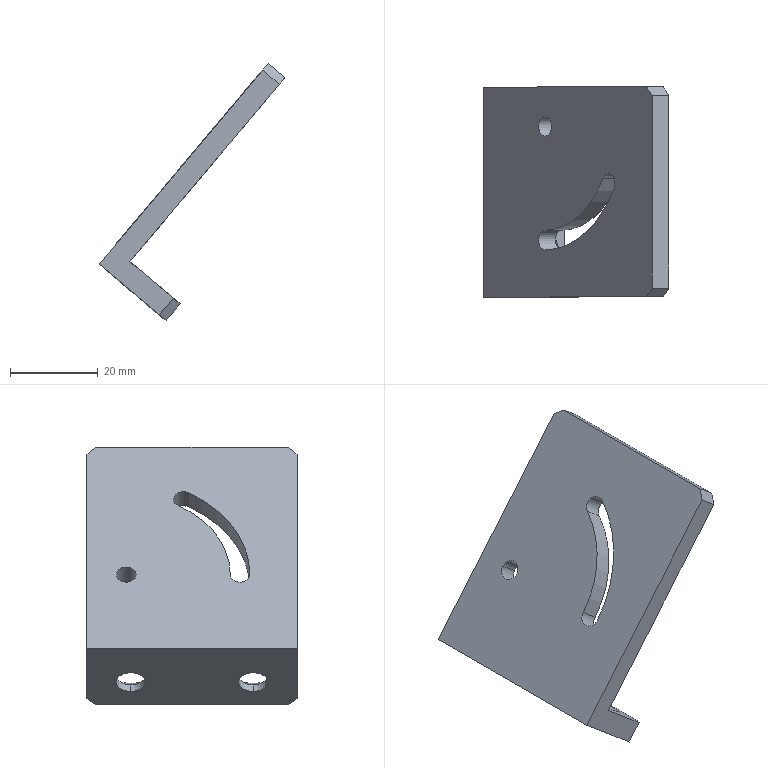Component | SolidWorks | 06CameraLightSourceMountPlate-1 | 1 solid | 26 faces | box 42.47 x 48 x 58.78 mm | volume 16585 mm3 | plane 12 | cylinder 10 | cone 4 | commonest cylinder face diameters 4.5 x4 6.6 x4 47.5 x1 56.5 x1 | material Aviation Aluminum-7075
build123d program:
from build123d import *

# Parameters (mm, degrees)
SKETCH1_W                                          = 48
SKETCH1_H                                          = 60
BOSS_EXTRUDE1_DEPTH                                = 5
SKETCH2_W                                          = 48
SKETCH2_H                                          = 5
BOSS_EXTRUDE2_DEPTH                                = 15
CHAMFER1_SIZE                                      = 2
HOLE_SIZE_ACCORDING_TO_TYPE_1_OF_HEXAG_D           = 6.6
HOLE_SIZE_ACCORDING_TO_TYPE_1_OF_HEXAG_DEPTH       = 15
HOLE_SIZE_ACCORDING_TO_TYPE_1_OF_HEXAG_CSINK_D     = 12.8
HOLE_SIZE_ACCORDING_TO_TYPE_1_OF_HEXAG_CSINK_ANGLE = 90
HOLE_SIZE_ACCORDING_TO_TYPE_1_OF_HEXAG_TIP         = 1.983
CUT_EXTRUDE1_REACH                                 = 43.243
SKETCH5_R                                          = 2.25
CUT_EXTRUDE2_REACH                                 = 43.243


with BuildPart() as part:
    # Sketch1 → Boss-Extrude1 (new body)
    with BuildSketch(Plane.XY):
        Rectangle(SKETCH1_W, SKETCH1_H)
    extrude(amount=BOSS_EXTRUDE1_DEPTH)

    # Sketch2 → Boss-Extrude2 (add)
    with BuildSketch(Plane.XY.offset(5)):
        with Locations((0, 27.5)):
            Rectangle(SKETCH2_W, SKETCH2_H)
    extrude(amount=BOSS_EXTRUDE2_DEPTH)

    # Chamfer1
    chamfer1_edges = [part.edges().sort_by_distance(p)[0] for p in [
        (-24, 27.5, 20),
        (24, 27.5, 20),
        (24, -30, 2.5),
        (-24, -30, 2.5),
    ]]
    chamfer(chamfer1_edges, length=CHAMFER1_SIZE)

    # Hole Size _According to_ Type 1 of Hexag
    with Locations(Plane(origin=(14, 25, 12), x_dir=(-1, 0, 0), z_dir=(0, -1, 0))):
        with Locations((0, 0), (28, 0)):
            CounterSinkHole(HOLE_SIZE_ACCORDING_TO_TYPE_1_OF_HEXAG_D / 2, HOLE_SIZE_ACCORDING_TO_TYPE_1_OF_HEXAG_CSINK_D / 2, depth=HOLE_SIZE_ACCORDING_TO_TYPE_1_OF_HEXAG_DEPTH, counter_sink_angle=HOLE_SIZE_ACCORDING_TO_TYPE_1_OF_HEXAG_CSINK_ANGLE)
            with Locations((0, 0, -(HOLE_SIZE_ACCORDING_TO_TYPE_1_OF_HEXAG_DEPTH + HOLE_SIZE_ACCORDING_TO_TYPE_1_OF_HEXAG_TIP / 2))):  # 118° drill point
                Cone(0, HOLE_SIZE_ACCORDING_TO_TYPE_1_OF_HEXAG_D / 2, HOLE_SIZE_ACCORDING_TO_TYPE_1_OF_HEXAG_TIP, mode=Mode.SUBTRACT)

    # Sketch5 → Cut-Extrude1 (cut, up to next)
    with BuildSketch(Plane.XY.offset(5), mode=Mode.PRIVATE) as cut_extrude1_sk1:
        with Locations((-15, 8)):
            Circle(SKETCH5_R)
    cut_extrude1_tool1 = extrude(cut_extrude1_sk1.sketch, amount=-CUT_EXTRUDE1_REACH, mode=Mode.PRIVATE) & part.part
    add(cut_extrude1_tool1.solids().sort_by_distance((-15, 8, 5))[0], mode=Mode.SUBTRACT)

    # Sketch6 → Cut-Extrude2 (cut, up to next)
    with BuildSketch(Plane.XY.offset(5), mode=Mode.PRIVATE) as cut_extrude2_sk1:
        with BuildLine():
            ThreePointArc((-0.875, -16.465), (9.465, -6.125), (13.25, 8))
            ThreePointArc((13.25, 8), (11, 10.25), (8.75, 8))
            ThreePointArc((8.75, 8), (5.568, -3.875), (-3.125, -12.568))
            ThreePointArc((-3.125, -12.568), (-3.949, -15.642), (-0.875, -16.465))
        make_face()
    cut_extrude2_tool1 = extrude(cut_extrude2_sk1.sketch, amount=-CUT_EXTRUDE2_REACH, mode=Mode.PRIVATE) & part.part
    add(cut_extrude2_tool1.solids().sort_by_distance((6.272, -4.281, 5))[0], mode=Mode.SUBTRACT)


solid = part.part

# Placed as in the assembly
solid = solid.moved(Location((-288.235, 173.645, -28.049), (180, 49.905, 90)))
STEP:
#1=CARTESIAN_POINT('',(-11.551,7.338,-1.345));
#2=VERTEX_POINT('',#1);
#3=CARTESIAN_POINT('',(-11.551,7.516,-1.345));
#4=VERTEX_POINT('',#3);
#5=CARTESIAN_POINT('',(-11.551,7.427,-1.345));
#6=DIRECTION('',(-0.765,-0.,0.6441));
#7=DIRECTION('',(0.,-1.,0.));
#8=AXIS2_PLACEMENT_3D('',#5,#6,#7);
#9=CIRCLE('',#8,0.08858);
#10=EDGE_CURVE('',#2,#4,#9,.T.);
#11=ORIENTED_EDGE('',*,*,#10,.T.);
#12=CARTESIAN_POINT('',(-11.4,7.516,-1.472));
#13=VERTEX_POINT('',#12);
#14=CARTESIAN_POINT('',(-11.551,7.516,-1.345));
#15=DIRECTION('',(0.765,0.,-0.6441));
#16=VECTOR('',#15,39.37);
#17=LINE('',#14,#16);
#18=EDGE_CURVE('',#4,#13,#17,.T.);
#19=ORIENTED_EDGE('',*,*,#18,.T.);
#20=CARTESIAN_POINT('',(-11.4,7.338,-1.472));
#21=VERTEX_POINT('',#20);
#22=CARTESIAN_POINT('',(-11.4,7.427,-1.472));
#23=DIRECTION('',(0.765,0.,-0.6441));
#24=DIRECTION('',(0.,-1.,0.));
#25=AXIS2_PLACEMENT_3D('',#22,#23,#24);
#26=CIRCLE('',#25,0.08858);
#27=EDGE_CURVE('',#13,#21,#26,.T.);
#28=ORIENTED_EDGE('',*,*,#27,.T.);
#29=CARTESIAN_POINT('',(-11.551,7.338,-1.345));
#30=DIRECTION('',(0.765,0.,-0.6441));
#31=VECTOR('',#30,39.37);
#32=LINE('',#29,#31);
#33=EDGE_CURVE('',#2,#21,#32,.T.);
#34=ORIENTED_EDGE('',*,*,#33,.F.);
#35=EDGE_LOOP('',(#11,#19,#28,#34));
#36=FACE_OUTER_BOUND('',#35,.T.);
#37=CARTESIAN_POINT('',(-11.551,7.427,-1.345));
#38=DIRECTION('',(0.765,0.,-0.6441));
#39=DIRECTION('',(0.,-1.,0.));
#40=AXIS2_PLACEMENT_3D('',#37,#38,#39);
#41=CYLINDRICAL_SURFACE('',#40,0.08858);
#42=ADVANCED_FACE('',(#36),#41,.F.);
#43=CARTESIAN_POINT('',(-11.6,6.285,-2.339));
#44=VERTEX_POINT('',#43);
#45=CARTESIAN_POINT('',(-11.798,6.285,-2.171));
#46=VERTEX_POINT('',#45);
#47=CARTESIAN_POINT('',(-11.699,6.285,-2.255));
#48=DIRECTION('',(0.6441,-0.,0.765));
#49=DIRECTION('',(-0.765,0.,0.6441));
#50=AXIS2_PLACEMENT_3D('',#47,#48,#49);
#51=CIRCLE('',#50,0.1299);
#52=EDGE_CURVE('',#44,#46,#51,.T.);
#53=ORIENTED_EDGE('',*,*,#52,.F.);
#54=CARTESIAN_POINT('',(-11.428,6.285,-2.324));
#55=VERTEX_POINT('',#54);
#56=CARTESIAN_POINT('',(-11.428,6.285,-2.324));
#57=DIRECTION('',(0.9963,-0.,0.0855));
#58=VECTOR('',#57,39.37);
#59=LINE('',#56,#58);
#60=EDGE_CURVE('',#44,#55,#59,.T.);
#61=ORIENTED_EDGE('',*,*,#60,.T.);
#62=CARTESIAN_POINT('',(-11.813,6.285,-1.999));
#63=VERTEX_POINT('',#62);
#64=CARTESIAN_POINT('',(-11.62,6.285,-2.161));
#65=DIRECTION('',(0.6441,-0.,0.765));
#66=DIRECTION('',(-0.765,0.,0.6441));
#67=AXIS2_PLACEMENT_3D('',#64,#65,#66);
#68=CIRCLE('',#67,0.252);
#69=EDGE_CURVE('',#55,#63,#68,.T.);
#70=ORIENTED_EDGE('',*,*,#69,.T.);
#71=CARTESIAN_POINT('',(-11.813,6.285,-1.999));
#72=DIRECTION('',(-0.0855,-0.,0.9963));
#73=VECTOR('',#72,39.37);
#74=LINE('',#71,#73);
#75=EDGE_CURVE('',#46,#63,#74,.T.);
#76=ORIENTED_EDGE('',*,*,#75,.F.);
#77=EDGE_LOOP('',(#53,#61,#70,#76));
#78=FACE_OUTER_BOUND('',#77,.T.);
#79=CARTESIAN_POINT('',(-11.62,6.285,-2.161));
#80=DIRECTION('',(0.6441,-0.,0.765));
#81=DIRECTION('',(-0.765,0.,0.6441));
#82=AXIS2_PLACEMENT_3D('',#79,#80,#81);
#83=CONICAL_SURFACE('',#82,0.252,0.7854);
#84=ADVANCED_FACE('',(#78),#83,.F.);
#85=CARTESIAN_POINT('',(-11.648,6.285,-2.396));
#86=VERTEX_POINT('',#85);
#87=CARTESIAN_POINT('',(-11.847,6.285,-2.228));
#88=VERTEX_POINT('',#87);
#89=CARTESIAN_POINT('',(-11.747,6.285,-2.312));
#90=DIRECTION('',(0.6441,-0.,0.765));
#91=DIRECTION('',(0.,-1.,-0.));
#92=AXIS2_PLACEMENT_3D('',#89,#90,#91);
#93=CIRCLE('',#92,0.1299);
#94=EDGE_CURVE('',#86,#88,#93,.T.);
#95=ORIENTED_EDGE('',*,*,#94,.F.);
#96=CARTESIAN_POINT('',(-11.521,6.285,-2.245));
#97=DIRECTION('',(0.6441,-0.,0.765));
#98=VECTOR('',#97,39.37);
#99=LINE('',#96,#98);
#100=EDGE_CURVE('',#86,#44,#99,.T.);
#101=ORIENTED_EDGE('',*,*,#100,.T.);
#102=ORIENTED_EDGE('',*,*,#52,.T.);
#103=CARTESIAN_POINT('',(-11.72,6.285,-2.078));
#104=DIRECTION('',(0.6441,-0.,0.765));
#105=VECTOR('',#104,39.37);
#106=LINE('',#103,#105);
#107=EDGE_CURVE('',#88,#46,#106,.T.);
#108=ORIENTED_EDGE('',*,*,#107,.F.);
#109=EDGE_LOOP('',(#95,#101,#102,#108));
#110=FACE_OUTER_BOUND('',#109,.T.);
#111=CARTESIAN_POINT('',(-11.62,6.285,-2.161));
#112=DIRECTION('',(0.6441,-0.,0.765));
#113=DIRECTION('',(-0.765,0.,0.6441));
#114=AXIS2_PLACEMENT_3D('',#111,#112,#113);
#115=CYLINDRICAL_SURFACE('',#114,0.1299);
#116=ADVANCED_FACE('',(#110),#115,.F.);
#117=CARTESIAN_POINT('',(-11.6,7.388,-2.339));
#118=VERTEX_POINT('',#117);
#119=CARTESIAN_POINT('',(-11.798,7.388,-2.171));
#120=VERTEX_POINT('',#119);
#121=CARTESIAN_POINT('',(-11.699,7.388,-2.255));
#122=DIRECTION('',(0.6441,-0.,0.765));
#123=DIRECTION('',(-0.765,0.,0.6441));
#124=AXIS2_PLACEMENT_3D('',#121,#122,#123);
#125=CIRCLE('',#124,0.1299);
#126=EDGE_CURVE('',#118,#120,#125,.T.);
#127=ORIENTED_EDGE('',*,*,#126,.F.);
#128=CARTESIAN_POINT('',(-11.428,7.388,-2.324));
#129=VERTEX_POINT('',#128);
#130=CARTESIAN_POINT('',(-11.428,7.388,-2.324));
#131=DIRECTION('',(0.9963,-0.,0.0855));
#132=VECTOR('',#131,39.37);
#133=LINE('',#130,#132);
#134=EDGE_CURVE('',#118,#129,#133,.T.);
#135=ORIENTED_EDGE('',*,*,#134,.T.);
#136=CARTESIAN_POINT('',(-11.813,7.388,-1.999));
#137=VERTEX_POINT('',#136);
#138=CARTESIAN_POINT('',(-11.62,7.388,-2.161));
#139=DIRECTION('',(0.6441,-0.,0.765));
#140=DIRECTION('',(-0.765,0.,0.6441));
#141=AXIS2_PLACEMENT_3D('',#138,#139,#140);
#142=CIRCLE('',#141,0.252);
#143=EDGE_CURVE('',#129,#137,#142,.T.);
#144=ORIENTED_EDGE('',*,*,#143,.T.);
#145=CARTESIAN_POINT('',(-11.813,7.388,-1.999));
#146=DIRECTION('',(-0.0855,-0.,0.9963));
#147=VECTOR('',#146,39.37);
#148=LINE('',#145,#147);
#149=EDGE_CURVE('',#120,#137,#148,.T.);
#150=ORIENTED_EDGE('',*,*,#149,.F.);
#151=EDGE_LOOP('',(#127,#135,#144,#150));
#152=FACE_OUTER_BOUND('',#151,.T.);
#153=CARTESIAN_POINT('',(-11.62,7.388,-2.161));
#154=DIRECTION('',(0.6441,-0.,0.765));
#155=DIRECTION('',(-0.765,0.,0.6441));
#156=AXIS2_PLACEMENT_3D('',#153,#154,#155);
#157=CONICAL_SURFACE('',#156,0.252,0.7854);
#158=ADVANCED_FACE('',(#152),#157,.F.);
#159=CARTESIAN_POINT('',(-11.648,7.388,-2.396));
#160=VERTEX_POINT('',#159);
#161=CARTESIAN_POINT('',(-11.847,7.388,-2.228));
#162=VERTEX_POINT('',#161);
#163=CARTESIAN_POINT('',(-11.747,7.388,-2.312));
#164=DIRECTION('',(0.6441,-0.,0.765));
#165=DIRECTION('',(0.,-1.,-0.));
#166=AXIS2_PLACEMENT_3D('',#163,#164,#165);
#167=CIRCLE('',#166,0.1299);
#168=EDGE_CURVE('',#160,#162,#167,.T.);
#169=ORIENTED_EDGE('',*,*,#168,.F.);
#170=CARTESIAN_POINT('',(-11.521,7.388,-2.245));
#171=DIRECTION('',(0.6441,-0.,0.765));
#172=VECTOR('',#171,39.37);
#173=LINE('',#170,#172);
#174=EDGE_CURVE('',#160,#118,#173,.T.);
#175=ORIENTED_EDGE('',*,*,#174,.T.);
#176=ORIENTED_EDGE('',*,*,#126,.T.);
#177=CARTESIAN_POINT('',(-11.72,7.388,-2.078));
#178=DIRECTION('',(0.6441,-0.,0.765));
#179=VECTOR('',#178,39.37);
#180=LINE('',#177,#179);
#181=EDGE_CURVE('',#162,#120,#180,.T.);
#182=ORIENTED_EDGE('',*,*,#181,.F.);
#183=EDGE_LOOP('',(#169,#175,#176,#182));
#184=FACE_OUTER_BOUND('',#183,.T.);
#185=CARTESIAN_POINT('',(-11.62,7.388,-2.161));
#186=DIRECTION('',(0.6441,-0.,0.765));
#187=DIRECTION('',(-0.765,0.,0.6441));
#188=AXIS2_PLACEMENT_3D('',#185,#186,#187);
#189=CYLINDRICAL_SURFACE('',#188,0.1299);
#190=ADVANCED_FACE('',(#184),#189,.F.);
#191=CARTESIAN_POINT('',(-11.44,7.781,-2.314));
#192=VERTEX_POINT('',#191);
#193=CARTESIAN_POINT('',(-11.831,7.781,-1.984));
#194=VERTEX_POINT('',#193);
#195=CARTESIAN_POINT('',(-11.379,7.781,-2.364));
#196=DIRECTION('',(-0.765,-0.,0.6441));
#197=VECTOR('',#196,39.37);
#198=LINE('',#195,#197);
#199=EDGE_CURVE('',#192,#194,#198,.T.);
#200=ORIENTED_EDGE('',*,*,#199,.F.);
#201=CARTESIAN_POINT('',(-11.566,7.781,-2.464));
#202=VERTEX_POINT('',#201);
#203=CARTESIAN_POINT('',(-11.566,7.781,-2.464));
#204=DIRECTION('',(-0.6441,0.,-0.765));
#205=VECTOR('',#204,39.37);
#206=LINE('',#203,#205);
#207=EDGE_CURVE('',#192,#202,#206,.T.);
#208=ORIENTED_EDGE('',*,*,#207,.T.);
#209=CARTESIAN_POINT('',(-12.109,7.781,-2.008));
#210=VERTEX_POINT('',#209);
#211=CARTESIAN_POINT('',(-11.958,7.781,-2.135));
#212=DIRECTION('',(-0.765,-0.,0.6441));
#213=VECTOR('',#212,39.37);
#214=LINE('',#211,#213);
#215=EDGE_CURVE('',#202,#210,#214,.T.);
#216=ORIENTED_EDGE('',*,*,#215,.T.);
#217=CARTESIAN_POINT('',(-10.638,7.781,-0.261));
#218=VERTEX_POINT('',#217);
#219=CARTESIAN_POINT('',(-10.587,7.781,-0.2008));
#220=DIRECTION('',(0.6441,-0.,0.765));
#221=VECTOR('',#220,39.37);
#222=LINE('',#219,#221);
#223=EDGE_CURVE('',#210,#218,#222,.T.);
#224=ORIENTED_EDGE('',*,*,#223,.T.);
#225=CARTESIAN_POINT('',(-10.487,7.781,-0.3878));
#226=VERTEX_POINT('',#225);
#227=CARTESIAN_POINT('',(-10.487,7.781,-0.3878));
#228=DIRECTION('',(0.765,0.,-0.6441));
#229=VECTOR('',#228,39.37);
#230=LINE('',#227,#229);
#231=EDGE_CURVE('',#218,#226,#230,.T.);
#232=ORIENTED_EDGE('',*,*,#231,.T.);
#233=CARTESIAN_POINT('',(-10.437,7.781,-0.3276));
#234=DIRECTION('',(0.6441,-0.,0.765));
#235=VECTOR('',#234,39.37);
#236=LINE('',#233,#235);
#237=EDGE_CURVE('',#194,#226,#236,.T.);
#238=ORIENTED_EDGE('',*,*,#237,.F.);
#239=EDGE_LOOP('',(#200,#208,#216,#224,#232,#238));
#240=FACE_OUTER_BOUND('',#239,.T.);
#241=CARTESIAN_POINT('',(-10.437,7.781,-0.3276));
#242=DIRECTION('',(-0.,-1.,-0.));
#243=DIRECTION('',(-0.6441,0.,-0.765));
#244=AXIS2_PLACEMENT_3D('',#241,#242,#243);
#245=PLANE('',#244);
#246=ADVANCED_FACE('',(#240),#245,.F.);
#247=CARTESIAN_POINT('',(-10.587,7.703,-0.2008));
#248=VERTEX_POINT('',#247);
#249=CARTESIAN_POINT('',(-10.587,5.97,-0.2008));
#250=VERTEX_POINT('',#249);
#251=CARTESIAN_POINT('',(-10.587,5.892,-0.2008));
#252=DIRECTION('',(-0.,-1.,-0.));
#253=VECTOR('',#252,39.37);
#254=LINE('',#251,#253);
#255=EDGE_CURVE('',#248,#250,#254,.T.);
#256=ORIENTED_EDGE('',*,*,#255,.T.);
#257=CARTESIAN_POINT('',(-10.437,5.97,-0.3276));
#258=VERTEX_POINT('',#257);
#259=CARTESIAN_POINT('',(-10.437,5.97,-0.3276));
#260=DIRECTION('',(0.765,0.,-0.6441));
#261=VECTOR('',#260,39.37);
#262=LINE('',#259,#261);
#263=EDGE_CURVE('',#250,#258,#262,.T.);
#264=ORIENTED_EDGE('',*,*,#263,.T.);
#265=CARTESIAN_POINT('',(-10.437,7.703,-0.3276));
#266=VERTEX_POINT('',#265);
#267=CARTESIAN_POINT('',(-10.437,5.892,-0.3276));
#268=DIRECTION('',(-0.,-1.,-0.));
#269=VECTOR('',#268,39.37);
#270=LINE('',#267,#269);
#271=EDGE_CURVE('',#266,#258,#270,.T.);
#272=ORIENTED_EDGE('',*,*,#271,.F.);
#273=CARTESIAN_POINT('',(-10.437,7.703,-0.3276));
#274=DIRECTION('',(-0.765,-0.,0.6441));
#275=VECTOR('',#274,39.37);
#276=LINE('',#273,#275);
#277=EDGE_CURVE('',#266,#248,#276,.T.);
#278=ORIENTED_EDGE('',*,*,#277,.T.);
#279=EDGE_LOOP('',(#256,#264,#272,#278));
#280=FACE_OUTER_BOUND('',#279,.T.);
#281=CARTESIAN_POINT('',(-10.437,5.892,-0.3276));
#282=DIRECTION('',(-0.6441,0.,-0.765));
#283=DIRECTION('',(0.,1.,0.));
#284=AXIS2_PLACEMENT_3D('',#281,#282,#283);
#285=PLANE('',#284);
#286=ADVANCED_FACE('',(#280),#285,.F.);
#287=CARTESIAN_POINT('',(-11.566,5.892,-2.464));
#288=VERTEX_POINT('',#287);
#289=CARTESIAN_POINT('',(-12.109,5.892,-2.008));
#290=VERTEX_POINT('',#289);
#291=CARTESIAN_POINT('',(-11.958,5.892,-2.135));
#292=DIRECTION('',(-0.765,-0.,0.6441));
#293=VECTOR('',#292,39.37);
#294=LINE('',#291,#293);
#295=EDGE_CURVE('',#288,#290,#294,.T.);
#296=ORIENTED_EDGE('',*,*,#295,.F.);
#297=CARTESIAN_POINT('',(-11.44,5.892,-2.314));
#298=VERTEX_POINT('',#297);
#299=CARTESIAN_POINT('',(-11.44,5.892,-2.314));
#300=DIRECTION('',(0.6441,-0.,0.765));
#301=VECTOR('',#300,39.37);
#302=LINE('',#299,#301);
#303=EDGE_CURVE('',#288,#298,#302,.T.);
#304=ORIENTED_EDGE('',*,*,#303,.T.);
#305=CARTESIAN_POINT('',(-11.831,5.892,-1.984));
#306=VERTEX_POINT('',#305);
#307=CARTESIAN_POINT('',(-11.379,5.892,-2.364));
#308=DIRECTION('',(-0.765,-0.,0.6441));
#309=VECTOR('',#308,39.37);
#310=LINE('',#307,#309);
#311=EDGE_CURVE('',#298,#306,#310,.T.);
#312=ORIENTED_EDGE('',*,*,#311,.T.);
#313=CARTESIAN_POINT('',(-10.487,5.892,-0.3878));
#314=VERTEX_POINT('',#313);
#315=CARTESIAN_POINT('',(-10.437,5.892,-0.3276));
#316=DIRECTION('',(-0.6441,0.,-0.765));
#317=VECTOR('',#316,39.37);
#318=LINE('',#315,#317);
#319=EDGE_CURVE('',#314,#306,#318,.T.);
#320=ORIENTED_EDGE('',*,*,#319,.F.);
#321=CARTESIAN_POINT('',(-10.638,5.892,-0.261));
#322=VERTEX_POINT('',#321);
#323=CARTESIAN_POINT('',(-10.487,5.892,-0.3878));
#324=DIRECTION('',(-0.765,-0.,0.6441));
#325=VECTOR('',#324,39.37);
#326=LINE('',#323,#325);
#327=EDGE_CURVE('',#314,#322,#326,.T.);
#328=ORIENTED_EDGE('',*,*,#327,.T.);
#329=CARTESIAN_POINT('',(-10.587,5.892,-0.2008));
#330=DIRECTION('',(-0.6441,0.,-0.765));
#331=VECTOR('',#330,39.37);
#332=LINE('',#329,#331);
#333=EDGE_CURVE('',#322,#290,#332,.T.);
#334=ORIENTED_EDGE('',*,*,#333,.T.);
#335=EDGE_LOOP('',(#296,#304,#312,#320,#328,#334));
#336=FACE_OUTER_BOUND('',#335,.T.);
#337=CARTESIAN_POINT('',(-10.437,5.892,-0.3276));
#338=DIRECTION('',(0.,1.,0.));
#339=DIRECTION('',(0.765,0.,-0.6441));
#340=AXIS2_PLACEMENT_3D('',#337,#338,#339);
#341=PLANE('',#340);
#342=ADVANCED_FACE('',(#336),#341,.F.);
#343=CARTESIAN_POINT('',(-11.747,6.285,-2.312));
#344=DIRECTION('',(0.6441,-0.,0.765));
#345=DIRECTION('',(0.,-1.,-0.));
#346=AXIS2_PLACEMENT_3D('',#343,#344,#345);
#347=CIRCLE('',#346,0.1299);
#348=EDGE_CURVE('',#88,#86,#347,.T.);
#349=ORIENTED_EDGE('',*,*,#348,.T.);
#350=ORIENTED_EDGE('',*,*,#94,.T.);
#351=EDGE_LOOP('',(#349,#350));
#352=FACE_BOUND('',#351,.T.);
#353=CARTESIAN_POINT('',(-11.747,7.388,-2.312));
#354=DIRECTION('',(0.6441,-0.,0.765));
#355=DIRECTION('',(0.,-1.,-0.));
#356=AXIS2_PLACEMENT_3D('',#353,#354,#355);
#357=CIRCLE('',#356,0.1299);
#358=EDGE_CURVE('',#162,#160,#357,.T.);
#359=ORIENTED_EDGE('',*,*,#358,.T.);
#360=ORIENTED_EDGE('',*,*,#168,.T.);
#361=EDGE_LOOP('',(#359,#360));
#362=FACE_BOUND('',#361,.T.);
#363=CARTESIAN_POINT('',(-11.506,5.97,-2.515));
#364=VERTEX_POINT('',#363);
#365=CARTESIAN_POINT('',(-11.506,7.703,-2.515));
#366=VERTEX_POINT('',#365);
#367=CARTESIAN_POINT('',(-11.506,5.892,-2.515));
#368=DIRECTION('',(0.,1.,0.));
#369=VECTOR('',#368,39.37);
#370=LINE('',#367,#369);
#371=EDGE_CURVE('',#364,#366,#370,.T.);
#372=ORIENTED_EDGE('',*,*,#371,.F.);
#373=CARTESIAN_POINT('',(-11.506,5.97,-2.515));
#374=DIRECTION('',(-0.5409,-0.7071,0.4554));
#375=VECTOR('',#374,39.37);
#376=LINE('',#373,#375);
#377=EDGE_CURVE('',#364,#288,#376,.T.);
#378=ORIENTED_EDGE('',*,*,#377,.T.);
#379=ORIENTED_EDGE('',*,*,#295,.T.);
#380=CARTESIAN_POINT('',(-12.109,5.892,-2.008));
#381=DIRECTION('',(0.,1.,0.));
#382=VECTOR('',#381,39.37);
#383=LINE('',#380,#382);
#384=EDGE_CURVE('',#290,#210,#383,.T.);
#385=ORIENTED_EDGE('',*,*,#384,.T.);
#386=ORIENTED_EDGE('',*,*,#215,.F.);
#387=CARTESIAN_POINT('',(-11.506,7.703,-2.515));
#388=DIRECTION('',(0.5409,-0.7071,-0.4554));
#389=VECTOR('',#388,39.37);
#390=LINE('',#387,#389);
#391=EDGE_CURVE('',#202,#366,#390,.T.);
#392=ORIENTED_EDGE('',*,*,#391,.T.);
#393=EDGE_LOOP('',(#372,#378,#379,#385,#386,#392));
#394=FACE_OUTER_BOUND('',#393,.T.);
#395=CARTESIAN_POINT('',(-11.958,5.892,-2.135));
#396=DIRECTION('',(0.6441,-0.,0.765));
#397=DIRECTION('',(-0.,-1.,-0.));
#398=AXIS2_PLACEMENT_3D('',#395,#396,#397);
#399=PLANE('',#398);
#400=ADVANCED_FACE('',(#352,#362,#394),#399,.F.);
#401=CARTESIAN_POINT('',(-10.879,6.959,-0.8526));
#402=VERTEX_POINT('',#401);
#403=CARTESIAN_POINT('',(-10.78,6.871,-0.7352));
#404=VERTEX_POINT('',#403);
#405=CARTESIAN_POINT('',(-10.829,6.915,-0.7939));
#406=DIRECTION('',(0.765,0.,-0.6441));
#407=DIRECTION('',(0.,-1.,-0.));
#408=AXIS2_PLACEMENT_3D('',#405,#406,#407);
#409=CIRCLE('',#408,0.08858);
#410=EDGE_CURVE('',#402,#404,#409,.T.);
#411=ORIENTED_EDGE('',*,*,#410,.F.);
#412=CARTESIAN_POINT('',(-11.4,6.492,-1.472));
#413=VERTEX_POINT('',#412);
#414=CARTESIAN_POINT('',(-11.4,7.427,-1.472));
#415=DIRECTION('',(-0.765,-0.,0.6441));
#416=DIRECTION('',(0.,-1.,-0.));
#417=AXIS2_PLACEMENT_3D('',#414,#415,#416);
#418=CIRCLE('',#417,0.935);
#419=EDGE_CURVE('',#413,#402,#418,.T.);
#420=ORIENTED_EDGE('',*,*,#419,.F.);
#421=CARTESIAN_POINT('',(-11.4,6.315,-1.472));
#422=VERTEX_POINT('',#421);
#423=CARTESIAN_POINT('',(-11.4,6.403,-1.472));
#424=DIRECTION('',(0.765,0.,-0.6441));
#425=DIRECTION('',(0.,-1.,0.));
#426=AXIS2_PLACEMENT_3D('',#423,#424,#425);
#427=CIRCLE('',#426,0.08858);
#428=EDGE_CURVE('',#422,#413,#427,.T.);
#429=ORIENTED_EDGE('',*,*,#428,.F.);
#430=CARTESIAN_POINT('',(-11.4,7.427,-1.472));
#431=DIRECTION('',(0.765,0.,-0.6441));
#432=DIRECTION('',(0.,-1.,-0.));
#433=AXIS2_PLACEMENT_3D('',#430,#431,#432);
#434=CIRCLE('',#433,1.112);
#435=EDGE_CURVE('',#404,#422,#434,.T.);
#436=ORIENTED_EDGE('',*,*,#435,.F.);
#437=EDGE_LOOP('',(#411,#420,#429,#436));
#438=FACE_BOUND('',#437,.T.);
#439=CARTESIAN_POINT('',(-11.4,7.427,-1.472));
#440=DIRECTION('',(0.765,0.,-0.6441));
#441=DIRECTION('',(0.,-1.,0.));
#442=AXIS2_PLACEMENT_3D('',#439,#440,#441);
#443=CIRCLE('',#442,0.08858);
#444=EDGE_CURVE('',#21,#13,#443,.T.);
#445=ORIENTED_EDGE('',*,*,#444,.F.);
#446=ORIENTED_EDGE('',*,*,#27,.F.);
#447=EDGE_LOOP('',(#445,#446));
#448=FACE_BOUND('',#447,.T.);
#449=ORIENTED_EDGE('',*,*,#271,.T.);
#450=CARTESIAN_POINT('',(-10.538,5.813,-0.448));
#451=DIRECTION('',(-0.4554,-0.7071,-0.5409));
#452=VECTOR('',#451,39.37);
#453=LINE('',#450,#452);
#454=EDGE_CURVE('',#258,#314,#453,.T.);
#455=ORIENTED_EDGE('',*,*,#454,.T.);
#456=ORIENTED_EDGE('',*,*,#319,.T.);
#457=CARTESIAN_POINT('',(-11.831,5.892,-1.984));
#458=DIRECTION('',(-0.,-1.,-0.));
#459=VECTOR('',#458,39.37);
#460=LINE('',#457,#459);
#461=EDGE_CURVE('',#194,#306,#460,.T.);
#462=ORIENTED_EDGE('',*,*,#461,.F.);
#463=ORIENTED_EDGE('',*,*,#237,.T.);
#464=CARTESIAN_POINT('',(-10.538,7.86,-0.448));
#465=DIRECTION('',(0.4554,-0.7071,0.5409));
#466=VECTOR('',#465,39.37);
#467=LINE('',#464,#466);
#468=EDGE_CURVE('',#226,#266,#467,.T.);
#469=ORIENTED_EDGE('',*,*,#468,.T.);
#470=EDGE_LOOP('',(#449,#455,#456,#462,#463,#469));
#471=FACE_OUTER_BOUND('',#470,.T.);
#472=CARTESIAN_POINT('',(-11.197,6.836,-1.231));
#473=DIRECTION('',(0.765,0.,-0.6441));
#474=DIRECTION('',(-0.,-1.,-0.));
#475=AXIS2_PLACEMENT_3D('',#472,#473,#474);
#476=PLANE('',#475);
#477=ADVANCED_FACE('',(#438,#448,#471),#476,.T.);
#478=CARTESIAN_POINT('',(-11.029,6.959,-0.7258));
#479=VERTEX_POINT('',#478);
#480=CARTESIAN_POINT('',(-11.551,6.492,-1.345));
#481=VERTEX_POINT('',#480);
#482=CARTESIAN_POINT('',(-11.551,7.427,-1.345));
#483=DIRECTION('',(0.765,0.,-0.6441));
#484=DIRECTION('',(0.,-1.,-0.));
#485=AXIS2_PLACEMENT_3D('',#482,#483,#484);
#486=CIRCLE('',#485,0.935);
#487=EDGE_CURVE('',#479,#481,#486,.T.);
#488=ORIENTED_EDGE('',*,*,#487,.F.);
#489=CARTESIAN_POINT('',(-10.93,6.871,-0.6084));
#490=VERTEX_POINT('',#489);
#491=CARTESIAN_POINT('',(-10.98,6.915,-0.6671));
#492=DIRECTION('',(-0.765,-0.,0.6441));
#493=DIRECTION('',(0.,-1.,-0.));
#494=AXIS2_PLACEMENT_3D('',#491,#492,#493);
#495=CIRCLE('',#494,0.08858);
#496=EDGE_CURVE('',#490,#479,#495,.T.);
#497=ORIENTED_EDGE('',*,*,#496,.F.);
#498=CARTESIAN_POINT('',(-11.551,6.315,-1.345));
#499=VERTEX_POINT('',#498);
#500=CARTESIAN_POINT('',(-11.551,7.427,-1.345));
#501=DIRECTION('',(-0.765,-0.,0.6441));
#502=DIRECTION('',(-0.,-1.,-0.));
#503=AXIS2_PLACEMENT_3D('',#500,#501,#502);
#504=CIRCLE('',#503,1.112);
#505=EDGE_CURVE('',#499,#490,#504,.T.);
#506=ORIENTED_EDGE('',*,*,#505,.F.);
#507=CARTESIAN_POINT('',(-11.551,6.403,-1.345));
#508=DIRECTION('',(-0.765,-0.,0.6441));
#509=DIRECTION('',(0.,-1.,-0.));
#510=AXIS2_PLACEMENT_3D('',#507,#508,#509);
#511=CIRCLE('',#510,0.08858);
#512=EDGE_CURVE('',#481,#499,#511,.T.);
#513=ORIENTED_EDGE('',*,*,#512,.F.);
#514=EDGE_LOOP('',(#488,#497,#506,#513));
#515=FACE_BOUND('',#514,.T.);
#516=ORIENTED_EDGE('',*,*,#10,.F.);
#517=CARTESIAN_POINT('',(-11.551,7.427,-1.345));
#518=DIRECTION('',(-0.765,-0.,0.6441));
#519=DIRECTION('',(0.,-1.,-0.));
#520=AXIS2_PLACEMENT_3D('',#517,#518,#519);
#521=CIRCLE('',#520,0.08858);
#522=EDGE_CURVE('',#4,#2,#521,.T.);
#523=ORIENTED_EDGE('',*,*,#522,.F.);
#524=EDGE_LOOP('',(#516,#523));
#525=FACE_BOUND('',#524,.T.);
#526=ORIENTED_EDGE('',*,*,#333,.F.);
#527=CARTESIAN_POINT('',(-10.638,5.892,-0.261));
#528=DIRECTION('',(0.4554,0.7071,0.5409));
#529=VECTOR('',#528,39.37);
#530=LINE('',#527,#529);
#531=EDGE_CURVE('',#322,#250,#530,.T.);
#532=ORIENTED_EDGE('',*,*,#531,.T.);
#533=ORIENTED_EDGE('',*,*,#255,.F.);
#534=CARTESIAN_POINT('',(-10.587,7.703,-0.2008));
#535=DIRECTION('',(-0.4554,0.7071,-0.5409));
#536=VECTOR('',#535,39.37);
#537=LINE('',#534,#536);
#538=EDGE_CURVE('',#248,#218,#537,.T.);
#539=ORIENTED_EDGE('',*,*,#538,.T.);
#540=ORIENTED_EDGE('',*,*,#223,.F.);
#541=ORIENTED_EDGE('',*,*,#384,.F.);
#542=EDGE_LOOP('',(#526,#532,#533,#539,#540,#541));
#543=FACE_OUTER_BOUND('',#542,.T.);
#544=CARTESIAN_POINT('',(-11.348,6.836,-1.104));
#545=DIRECTION('',(0.765,0.,-0.6441));
#546=DIRECTION('',(-0.,-1.,-0.));
#547=AXIS2_PLACEMENT_3D('',#544,#545,#546);
#548=PLANE('',#547);
#549=ADVANCED_FACE('',(#515,#525,#543),#548,.F.);
#550=CARTESIAN_POINT('',(-11.62,6.285,-2.161));
#551=DIRECTION('',(0.6441,-0.,0.765));
#552=DIRECTION('',(-0.765,0.,0.6441));
#553=AXIS2_PLACEMENT_3D('',#550,#551,#552);
#554=CIRCLE('',#553,0.252);
#555=EDGE_CURVE('',#63,#55,#554,.T.);
#556=ORIENTED_EDGE('',*,*,#555,.F.);
#557=ORIENTED_EDGE('',*,*,#69,.F.);
#558=EDGE_LOOP('',(#556,#557));
#559=FACE_BOUND('',#558,.T.);
#560=CARTESIAN_POINT('',(-11.62,7.388,-2.161));
#561=DIRECTION('',(0.6441,-0.,0.765));
#562=DIRECTION('',(-0.765,0.,0.6441));
#563=AXIS2_PLACEMENT_3D('',#560,#561,#562);
#564=CIRCLE('',#563,0.252);
#565=EDGE_CURVE('',#137,#129,#564,.T.);
#566=ORIENTED_EDGE('',*,*,#565,.F.);
#567=ORIENTED_EDGE('',*,*,#143,.F.);
#568=EDGE_LOOP('',(#566,#567));
#569=FACE_BOUND('',#568,.T.);
#570=ORIENTED_EDGE('',*,*,#311,.F.);
#571=CARTESIAN_POINT('',(-11.379,5.97,-2.364));
#572=VERTEX_POINT('',#571);
#573=CARTESIAN_POINT('',(-11.379,5.97,-2.364));
#574=DIRECTION('',(0.5409,0.7071,-0.4554));
#575=VECTOR('',#574,39.37);
#576=LINE('',#573,#575);
#577=EDGE_CURVE('',#298,#572,#576,.T.);
#578=ORIENTED_EDGE('',*,*,#577,.T.);
#579=CARTESIAN_POINT('',(-11.379,7.703,-2.364));
#580=VERTEX_POINT('',#579);
#581=CARTESIAN_POINT('',(-11.379,5.892,-2.364));
#582=DIRECTION('',(-0.,-1.,-0.));
#583=VECTOR('',#582,39.37);
#584=LINE('',#581,#583);
#585=EDGE_CURVE('',#580,#572,#584,.T.);
#586=ORIENTED_EDGE('',*,*,#585,.F.);
#587=CARTESIAN_POINT('',(-11.379,7.703,-2.364));
#588=DIRECTION('',(-0.5409,0.7071,0.4554));
#589=VECTOR('',#588,39.37);
#590=LINE('',#587,#589);
#591=EDGE_CURVE('',#580,#192,#590,.T.);
#592=ORIENTED_EDGE('',*,*,#591,.T.);
#593=ORIENTED_EDGE('',*,*,#199,.T.);
#594=ORIENTED_EDGE('',*,*,#461,.T.);
#595=EDGE_LOOP('',(#570,#578,#586,#592,#593,#594));
#596=FACE_OUTER_BOUND('',#595,.T.);
#597=CARTESIAN_POINT('',(-11.379,5.892,-2.364));
#598=DIRECTION('',(-0.6441,0.,-0.765));
#599=DIRECTION('',(0.,1.,0.));
#600=AXIS2_PLACEMENT_3D('',#597,#598,#599);
#601=PLANE('',#600);
#602=ADVANCED_FACE('',(#559,#569,#596),#601,.F.);
#603=ORIENTED_EDGE('',*,*,#585,.T.);
#604=CARTESIAN_POINT('',(-11.506,5.97,-2.515));
#605=DIRECTION('',(-0.6441,0.,-0.765));
#606=VECTOR('',#605,39.37);
#607=LINE('',#604,#606);
#608=EDGE_CURVE('',#572,#364,#607,.T.);
#609=ORIENTED_EDGE('',*,*,#608,.T.);
#610=ORIENTED_EDGE('',*,*,#371,.T.);
#611=CARTESIAN_POINT('',(-11.379,7.703,-2.364));
#612=DIRECTION('',(0.6441,-0.,0.765));
#613=VECTOR('',#612,39.37);
#614=LINE('',#611,#613);
#615=EDGE_CURVE('',#366,#580,#614,.T.);
#616=ORIENTED_EDGE('',*,*,#615,.T.);
#617=EDGE_LOOP('',(#603,#609,#610,#616));
#618=FACE_OUTER_BOUND('',#617,.T.);
#619=CARTESIAN_POINT('',(-10.745,6.836,-1.611));
#620=DIRECTION('',(0.765,0.,-0.6441));
#621=DIRECTION('',(-0.,-1.,-0.));
#622=AXIS2_PLACEMENT_3D('',#619,#620,#621);
#623=PLANE('',#622);
#624=ADVANCED_FACE('',(#618),#623,.T.);
#625=ORIENTED_EDGE('',*,*,#577,.F.);
#626=ORIENTED_EDGE('',*,*,#303,.F.);
#627=ORIENTED_EDGE('',*,*,#377,.F.);
#628=ORIENTED_EDGE('',*,*,#608,.F.);
#629=EDGE_LOOP('',(#625,#626,#627,#628));
#630=FACE_OUTER_BOUND('',#629,.T.);
#631=CARTESIAN_POINT('',(-10.745,5.97,-1.611));
#632=DIRECTION('',(0.5409,-0.7071,-0.4554));
#633=DIRECTION('',(0.6441,-0.,0.765));
#634=AXIS2_PLACEMENT_3D('',#631,#632,#633);
#635=PLANE('',#634);
#636=ADVANCED_FACE('',(#630),#635,.T.);
#637=ORIENTED_EDGE('',*,*,#391,.F.);
#638=ORIENTED_EDGE('',*,*,#207,.F.);
#639=ORIENTED_EDGE('',*,*,#591,.F.);
#640=ORIENTED_EDGE('',*,*,#615,.F.);
#641=EDGE_LOOP('',(#637,#638,#639,#640));
#642=FACE_OUTER_BOUND('',#641,.T.);
#643=CARTESIAN_POINT('',(-10.745,7.703,-1.611));
#644=DIRECTION('',(0.5409,0.7071,-0.4554));
#645=DIRECTION('',(-0.6441,0.,-0.765));
#646=AXIS2_PLACEMENT_3D('',#643,#644,#645);
#647=PLANE('',#646);
#648=ADVANCED_FACE('',(#642),#647,.T.);
#649=ORIENTED_EDGE('',*,*,#454,.F.);
#650=ORIENTED_EDGE('',*,*,#263,.F.);
#651=ORIENTED_EDGE('',*,*,#531,.F.);
#652=ORIENTED_EDGE('',*,*,#327,.F.);
#653=EDGE_LOOP('',(#649,#650,#651,#652));
#654=FACE_OUTER_BOUND('',#653,.T.);
#655=CARTESIAN_POINT('',(-10.487,5.892,-0.3878));
#656=DIRECTION('',(-0.4554,0.7071,-0.5409));
#657=DIRECTION('',(-0.765,-0.,0.6441));
#658=AXIS2_PLACEMENT_3D('',#655,#656,#657);
#659=PLANE('',#658);
#660=ADVANCED_FACE('',(#654),#659,.F.);
#661=ORIENTED_EDGE('',*,*,#468,.F.);
#662=ORIENTED_EDGE('',*,*,#231,.F.);
#663=ORIENTED_EDGE('',*,*,#538,.F.);
#664=ORIENTED_EDGE('',*,*,#277,.F.);
#665=EDGE_LOOP('',(#661,#662,#663,#664));
#666=FACE_OUTER_BOUND('',#665,.T.);
#667=CARTESIAN_POINT('',(-10.437,7.703,-0.3276));
#668=DIRECTION('',(-0.4554,-0.7071,-0.5409));
#669=DIRECTION('',(-0.765,-0.,0.6441));
#670=AXIS2_PLACEMENT_3D('',#667,#668,#669);
#671=PLANE('',#670);
#672=ADVANCED_FACE('',(#666),#671,.F.);
#673=ORIENTED_EDGE('',*,*,#174,.F.);
#674=ORIENTED_EDGE('',*,*,#358,.F.);
#675=ORIENTED_EDGE('',*,*,#181,.T.);
#676=CARTESIAN_POINT('',(-11.699,7.388,-2.255));
#677=DIRECTION('',(0.6441,-0.,0.765));
#678=DIRECTION('',(-0.765,0.,0.6441));
#679=AXIS2_PLACEMENT_3D('',#676,#677,#678);
#680=CIRCLE('',#679,0.1299);
#681=EDGE_CURVE('',#120,#118,#680,.T.);
#682=ORIENTED_EDGE('',*,*,#681,.T.);
#683=EDGE_LOOP('',(#673,#674,#675,#682));
#684=FACE_OUTER_BOUND('',#683,.T.);
#685=CARTESIAN_POINT('',(-11.62,7.388,-2.161));
#686=DIRECTION('',(0.6441,-0.,0.765));
#687=DIRECTION('',(-0.765,0.,0.6441));
#688=AXIS2_PLACEMENT_3D('',#685,#686,#687);
#689=CYLINDRICAL_SURFACE('',#688,0.1299);
#690=ADVANCED_FACE('',(#684),#689,.F.);
#691=ORIENTED_EDGE('',*,*,#134,.F.);
#692=ORIENTED_EDGE('',*,*,#681,.F.);
#693=ORIENTED_EDGE('',*,*,#149,.T.);
#694=ORIENTED_EDGE('',*,*,#565,.T.);
#695=EDGE_LOOP('',(#691,#692,#693,#694));
#696=FACE_OUTER_BOUND('',#695,.T.);
#697=CARTESIAN_POINT('',(-11.62,7.388,-2.161));
#698=DIRECTION('',(0.6441,-0.,0.765));
#699=DIRECTION('',(-0.765,0.,0.6441));
#700=AXIS2_PLACEMENT_3D('',#697,#698,#699);
#701=CONICAL_SURFACE('',#700,0.252,0.7854);
#702=ADVANCED_FACE('',(#696),#701,.F.);
#703=ORIENTED_EDGE('',*,*,#100,.F.);
#704=ORIENTED_EDGE('',*,*,#348,.F.);
#705=ORIENTED_EDGE('',*,*,#107,.T.);
#706=CARTESIAN_POINT('',(-11.699,6.285,-2.255));
#707=DIRECTION('',(0.6441,-0.,0.765));
#708=DIRECTION('',(-0.765,0.,0.6441));
#709=AXIS2_PLACEMENT_3D('',#706,#707,#708);
#710=CIRCLE('',#709,0.1299);
#711=EDGE_CURVE('',#46,#44,#710,.T.);
#712=ORIENTED_EDGE('',*,*,#711,.T.);
#713=EDGE_LOOP('',(#703,#704,#705,#712));
#714=FACE_OUTER_BOUND('',#713,.T.);
#715=CARTESIAN_POINT('',(-11.62,6.285,-2.161));
#716=DIRECTION('',(0.6441,-0.,0.765));
#717=DIRECTION('',(-0.765,0.,0.6441));
#718=AXIS2_PLACEMENT_3D('',#715,#716,#717);
#719=CYLINDRICAL_SURFACE('',#718,0.1299);
#720=ADVANCED_FACE('',(#714),#719,.F.);
#721=ORIENTED_EDGE('',*,*,#60,.F.);
#722=ORIENTED_EDGE('',*,*,#711,.F.);
#723=ORIENTED_EDGE('',*,*,#75,.T.);
#724=ORIENTED_EDGE('',*,*,#555,.T.);
#725=EDGE_LOOP('',(#721,#722,#723,#724));
#726=FACE_OUTER_BOUND('',#725,.T.);
#727=CARTESIAN_POINT('',(-11.62,6.285,-2.161));
#728=DIRECTION('',(0.6441,-0.,0.765));
#729=DIRECTION('',(-0.765,0.,0.6441));
#730=AXIS2_PLACEMENT_3D('',#727,#728,#729);
#731=CONICAL_SURFACE('',#730,0.252,0.7854);
#732=ADVANCED_FACE('',(#726),#731,.F.);
#733=ORIENTED_EDGE('',*,*,#18,.F.);
#734=ORIENTED_EDGE('',*,*,#522,.T.);
#735=ORIENTED_EDGE('',*,*,#33,.T.);
#736=ORIENTED_EDGE('',*,*,#444,.T.);
#737=EDGE_LOOP('',(#733,#734,#735,#736));
#738=FACE_OUTER_BOUND('',#737,.T.);
#739=CARTESIAN_POINT('',(-11.551,7.427,-1.345));
#740=DIRECTION('',(0.765,0.,-0.6441));
#741=DIRECTION('',(0.,-1.,0.));
#742=AXIS2_PLACEMENT_3D('',#739,#740,#741);
#743=CYLINDRICAL_SURFACE('',#742,0.08858);
#744=ADVANCED_FACE('',(#738),#743,.F.);
#745=ORIENTED_EDGE('',*,*,#496,.T.);
#746=CARTESIAN_POINT('',(-11.029,6.959,-0.7257));
#747=DIRECTION('',(0.765,0.,-0.6441));
#748=VECTOR('',#747,39.37);
#749=LINE('',#746,#748);
#750=EDGE_CURVE('',#479,#402,#749,.T.);
#751=ORIENTED_EDGE('',*,*,#750,.T.);
#752=ORIENTED_EDGE('',*,*,#410,.T.);
#753=CARTESIAN_POINT('',(-10.93,6.871,-0.6084));
#754=DIRECTION('',(0.765,0.,-0.6441));
#755=VECTOR('',#754,39.37);
#756=LINE('',#753,#755);
#757=EDGE_CURVE('',#490,#404,#756,.T.);
#758=ORIENTED_EDGE('',*,*,#757,.F.);
#759=EDGE_LOOP('',(#745,#751,#752,#758));
#760=FACE_OUTER_BOUND('',#759,.T.);
#761=CARTESIAN_POINT('',(-10.98,6.915,-0.6671));
#762=DIRECTION('',(0.765,0.,-0.6441));
#763=DIRECTION('',(0.,-1.,-0.));
#764=AXIS2_PLACEMENT_3D('',#761,#762,#763);
#765=CYLINDRICAL_SURFACE('',#764,0.08858);
#766=ADVANCED_FACE('',(#760),#765,.F.);
#767=ORIENTED_EDGE('',*,*,#487,.T.);
#768=CARTESIAN_POINT('',(-11.551,6.492,-1.345));
#769=DIRECTION('',(0.765,0.,-0.6441));
#770=VECTOR('',#769,39.37);
#771=LINE('',#768,#770);
#772=EDGE_CURVE('',#481,#413,#771,.T.);
#773=ORIENTED_EDGE('',*,*,#772,.T.);
#774=ORIENTED_EDGE('',*,*,#419,.T.);
#775=ORIENTED_EDGE('',*,*,#750,.F.);
#776=EDGE_LOOP('',(#767,#773,#774,#775));
#777=FACE_OUTER_BOUND('',#776,.T.);
#778=CARTESIAN_POINT('',(-11.551,7.427,-1.345));
#779=DIRECTION('',(0.765,0.,-0.6441));
#780=DIRECTION('',(0.,-1.,-0.));
#781=AXIS2_PLACEMENT_3D('',#778,#779,#780);
#782=CYLINDRICAL_SURFACE('',#781,0.935);
#783=ADVANCED_FACE('',(#777),#782,.T.);
#784=ORIENTED_EDGE('',*,*,#512,.T.);
#785=CARTESIAN_POINT('',(-11.551,6.315,-1.345));
#786=DIRECTION('',(0.765,0.,-0.6441));
#787=VECTOR('',#786,39.37);
#788=LINE('',#785,#787);
#789=EDGE_CURVE('',#499,#422,#788,.T.);
#790=ORIENTED_EDGE('',*,*,#789,.T.);
#791=ORIENTED_EDGE('',*,*,#428,.T.);
#792=ORIENTED_EDGE('',*,*,#772,.F.);
#793=EDGE_LOOP('',(#784,#790,#791,#792));
#794=FACE_OUTER_BOUND('',#793,.T.);
#795=CARTESIAN_POINT('',(-11.551,6.403,-1.345));
#796=DIRECTION('',(0.765,0.,-0.6441));
#797=DIRECTION('',(0.,-1.,0.));
#798=AXIS2_PLACEMENT_3D('',#795,#796,#797);
#799=CYLINDRICAL_SURFACE('',#798,0.08858);
#800=ADVANCED_FACE('',(#794),#799,.F.);
#801=ORIENTED_EDGE('',*,*,#505,.T.);
#802=ORIENTED_EDGE('',*,*,#757,.T.);
#803=ORIENTED_EDGE('',*,*,#435,.T.);
#804=ORIENTED_EDGE('',*,*,#789,.F.);
#805=EDGE_LOOP('',(#801,#802,#803,#804));
#806=FACE_OUTER_BOUND('',#805,.T.);
#807=CARTESIAN_POINT('',(-11.551,7.427,-1.345));
#808=DIRECTION('',(0.765,0.,-0.6441));
#809=DIRECTION('',(0.,-1.,-0.));
#810=AXIS2_PLACEMENT_3D('',#807,#808,#809);
#811=CYLINDRICAL_SURFACE('',#810,1.112);
#812=ADVANCED_FACE('',(#806),#811,.F.);
#813=CLOSED_SHELL('',(#42,#84,#116,#158,#190,#246,#286,#342,#400,#477,#549,#602,#624,#636,#648,#660,#672,#690,#702,#720,#732,#744,#766,#783,#800,#812));
#814=MANIFOLD_SOLID_BREP('',#813);
#815=CARTESIAN_POINT('',(0.,0.,0.));
#816=DIRECTION('',(0.,0.,1.));
#817=DIRECTION('',(1.,0.,0.));
#818=AXIS2_PLACEMENT_3D('',#815,#816,#817);
#819=(LENGTH_UNIT()NAMED_UNIT(*)SI_UNIT($,.METRE.));
#820=LENGTH_MEASURE_WITH_UNIT(LENGTH_MEASURE(0.0254),#819);
#821=DIMENSIONAL_EXPONENTS(1.,0.,0.,0.,0.,0.,0.);
#822=(CONVERSION_BASED_UNIT('',#820)LENGTH_UNIT()NAMED_UNIT(#821));
#823=UNCERTAINTY_MEASURE_WITH_UNIT(LENGTH_MEASURE(0.00001),#822,'','');
#824=(NAMED_UNIT(*)PLANE_ANGLE_UNIT()SI_UNIT($,.RADIAN.));
#825=(NAMED_UNIT(*)SI_UNIT($,.STERADIAN.)SOLID_ANGLE_UNIT());
#826=(GEOMETRIC_REPRESENTATION_CONTEXT(3)GLOBAL_UNCERTAINTY_ASSIGNED_CONTEXT((#823))GLOBAL_UNIT_ASSIGNED_CONTEXT((#822,#824,#825))REPRESENTATION_CONTEXT('',''));
#827=ADVANCED_BREP_SHAPE_REPRESENTATION('',(#814,#818),#826);
#828=COLOUR_RGB('',0.7922,0.8196,0.9333);
#829=FILL_AREA_STYLE_COLOUR('',#828);
#830=FILL_AREA_STYLE('',(#829));
#831=SURFACE_STYLE_FILL_AREA(#830);
#832=SURFACE_SIDE_STYLE('',(#831));
#833=SURFACE_STYLE_USAGE(.BOTH.,#832);
#834=PRESENTATION_STYLE_ASSIGNMENT((#833));
#835=STYLED_ITEM('',(#834),#814);
#836=(LENGTH_UNIT()NAMED_UNIT(*)SI_UNIT($,.METRE.));
#837=LENGTH_MEASURE_WITH_UNIT(LENGTH_MEASURE(0.0254),#836);
#838=DIMENSIONAL_EXPONENTS(1.,0.,0.,0.,0.,0.,0.);
#839=(CONVERSION_BASED_UNIT('',#837)LENGTH_UNIT()NAMED_UNIT(#838));
#840=UNCERTAINTY_MEASURE_WITH_UNIT(LENGTH_MEASURE(0.00001),#839,'','');
#841=(NAMED_UNIT(*)PLANE_ANGLE_UNIT()SI_UNIT($,.RADIAN.));
#842=(NAMED_UNIT(*)SI_UNIT($,.STERADIAN.)SOLID_ANGLE_UNIT());
#843=(GEOMETRIC_REPRESENTATION_CONTEXT(3)GLOBAL_UNCERTAINTY_ASSIGNED_CONTEXT((#840))GLOBAL_UNIT_ASSIGNED_CONTEXT((#839,#841,#842))REPRESENTATION_CONTEXT('',''));
#844=MECHANICAL_DESIGN_GEOMETRIC_PRESENTATION_REPRESENTATION('',(#835),#843);
#845=PRESENTATION_LAYER_ASSIGNMENT('','',(#835));